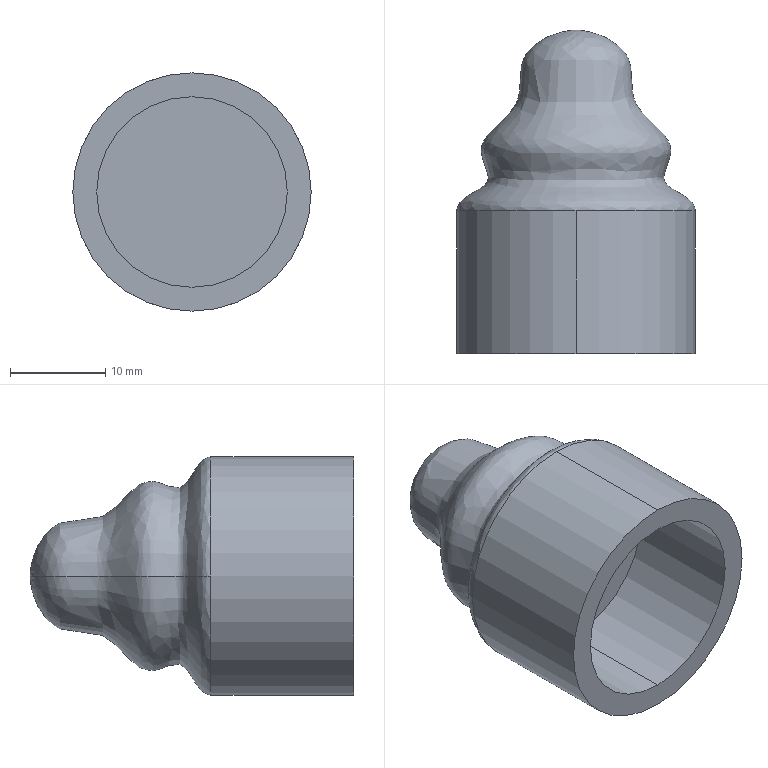Component | SolidWorks | TopCover-1 | 1 solid | 8 faces | box 25 x 33.95 x 25 mm | volume 7353 mm3 | cylinder 4 | spline 2 | plane 2 | commonest cylinder face diameters 20 x2 25 x2
build123d program:
from build123d import *

# Parameters (mm, degrees)
SKETCH1_R           = 12.5
BOSS_EXTRUDE1_DEPTH = 15
SHELL1_T            = -2.5


with BuildPart() as part:
    # Sketch1 → Boss-Extrude1 (new body)
    with BuildSketch(Plane(origin=(0, 0, 0), x_dir=(1, 0, 0), z_dir=(0, 1, 0))):
        with Locations(Location((0, 0, 0), (0, 0, 270))):
            Circle(SKETCH1_R)
    extrude(amount=BOSS_EXTRUDE1_DEPTH)

    # Shell1
    shell1_openings = [part.faces().sort_by_distance(p)[0] for p in [
        (0, 0, 0),
    ]]
    offset(amount=SHELL1_T, openings=shell1_openings, kind=Kind.INTERSECTION)

    # Sketch2 → Revolve1 (revolve)
    with BuildSketch(Plane.XY):
        with BuildLine():
            Line((-12.5, 15), (0, 15))
            Line((0, 15), (0, 33.954))
            add(Edge.make_bspline(
                [(-12.5, 15), (-12.5, 16.591), (-7.793, 17.261), (-11.573, 22.581), (-4.955, 25.26), (-6.75, 32.024), (-1.878, 33.951), (0, 33.954)],
                knots=[0, 0, 0, 0, 0.1825, 0.2981, 0.5567, 0.738, 1, 1, 1, 1], degree=3))
        make_face()
    revolve(axis=Axis((0, 15, 0), (0, 1, 0)))


solid = part.part

# Placed as in the assembly
solid = solid.moved(Location((155, 1577.501, -154.999), (0, 0, 0)))
STEP:
#1=CARTESIAN_POINT('',(6.102,63.443,-6.102));
#2=VERTEX_POINT('',#1);
#3=CARTESIAN_POINT('',(5.61,62.697,-6.102));
#4=VERTEX_POINT('',#3);
#5=CARTESIAN_POINT('',(6.102,63.443,-6.102));
#6=CARTESIAN_POINT('',(6.028,63.443,-6.102));
#7=CARTESIAN_POINT('',(5.837,63.367,-6.102));
#8=CARTESIAN_POINT('',(5.907,63.101,-6.102));
#9=CARTESIAN_POINT('',(5.647,62.995,-6.102));
#10=CARTESIAN_POINT('',(5.796,62.786,-6.102));
#11=CARTESIAN_POINT('',(5.61,62.759,-6.102));
#12=CARTESIAN_POINT('',(5.61,62.697,-6.102));
#13=B_SPLINE_CURVE_WITH_KNOTS('',3,(#5,#6,#7,#8,#9,#10,#11,#12),.UNSPECIFIED.,.F.,.F.,(4,1,1,1,1,4),(0.,0.262,0.4433,0.7019,0.8175,1.),.UNSPECIFIED.);
#14=EDGE_CURVE('',#2,#4,#13,.T.);
#15=ORIENTED_EDGE('',*,*,#14,.F.);
#16=CARTESIAN_POINT('',(6.594,62.697,-6.102));
#17=VERTEX_POINT('',#16);
#18=CARTESIAN_POINT('',(6.102,63.443,-6.102));
#19=CARTESIAN_POINT('',(6.176,63.443,-6.102));
#20=CARTESIAN_POINT('',(6.368,63.367,-6.102));
#21=CARTESIAN_POINT('',(6.297,63.101,-6.102));
#22=CARTESIAN_POINT('',(6.558,62.995,-6.102));
#23=CARTESIAN_POINT('',(6.409,62.786,-6.102));
#24=CARTESIAN_POINT('',(6.594,62.759,-6.102));
#25=CARTESIAN_POINT('',(6.594,62.697,-6.102));
#26=B_SPLINE_CURVE_WITH_KNOTS('',3,(#18,#19,#20,#21,#22,#23,#24,#25),.UNSPECIFIED.,.F.,.F.,(4,1,1,1,1,4),(0.,0.262,0.4433,0.7019,0.8175,1.),.UNSPECIFIED.);
#27=EDGE_CURVE('',#2,#17,#26,.T.);
#28=ORIENTED_EDGE('',*,*,#27,.T.);
#29=CARTESIAN_POINT('',(6.102,62.697,-6.594));
#30=VERTEX_POINT('',#29);
#31=CARTESIAN_POINT('',(6.102,62.697,-6.102));
#32=DIRECTION('',(0.,1.,0.));
#33=DIRECTION('',(0.,0.,1.));
#34=AXIS2_PLACEMENT_3D('',#31,#32,#33);
#35=CIRCLE('',#34,0.4921);
#36=EDGE_CURVE('',#17,#30,#35,.T.);
#37=ORIENTED_EDGE('',*,*,#36,.T.);
#38=CARTESIAN_POINT('',(6.102,62.697,-6.102));
#39=DIRECTION('',(0.,1.,0.));
#40=DIRECTION('',(0.,0.,1.));
#41=AXIS2_PLACEMENT_3D('',#38,#39,#40);
#42=CIRCLE('',#41,0.4921);
#43=EDGE_CURVE('',#30,#4,#42,.T.);
#44=ORIENTED_EDGE('',*,*,#43,.T.);
#45=EDGE_LOOP('',(#15,#28,#37,#44));
#46=FACE_OUTER_BOUND('',#45,.T.);
#47=CARTESIAN_POINT('',(6.102,63.443,-6.102));
#48=CARTESIAN_POINT('',(6.102,63.443,-6.102));
#49=CARTESIAN_POINT('',(6.102,63.443,-6.102));
#50=CARTESIAN_POINT('',(6.102,63.443,-6.102));
#51=CARTESIAN_POINT('',(6.028,63.443,-6.102));
#52=CARTESIAN_POINT('',(6.028,63.443,-6.25));
#53=CARTESIAN_POINT('',(6.176,63.443,-6.25));
#54=CARTESIAN_POINT('',(6.176,63.443,-6.102));
#55=CARTESIAN_POINT('',(5.837,63.367,-6.102));
#56=CARTESIAN_POINT('',(5.837,63.367,-6.634));
#57=CARTESIAN_POINT('',(6.368,63.367,-6.634));
#58=CARTESIAN_POINT('',(6.368,63.367,-6.102));
#59=CARTESIAN_POINT('',(5.907,63.101,-6.102));
#60=CARTESIAN_POINT('',(5.907,63.101,-6.492));
#61=CARTESIAN_POINT('',(6.297,63.101,-6.492));
#62=CARTESIAN_POINT('',(6.297,63.101,-6.102));
#63=CARTESIAN_POINT('',(5.647,62.995,-6.102));
#64=CARTESIAN_POINT('',(5.647,62.995,-7.014));
#65=CARTESIAN_POINT('',(6.558,62.995,-7.014));
#66=CARTESIAN_POINT('',(6.558,62.995,-6.102));
#67=CARTESIAN_POINT('',(5.796,62.786,-6.102));
#68=CARTESIAN_POINT('',(5.796,62.786,-6.716));
#69=CARTESIAN_POINT('',(6.409,62.786,-6.716));
#70=CARTESIAN_POINT('',(6.409,62.786,-6.102));
#71=CARTESIAN_POINT('',(5.61,62.759,-6.102));
#72=CARTESIAN_POINT('',(5.61,62.759,-7.087));
#73=CARTESIAN_POINT('',(6.594,62.759,-7.087));
#74=CARTESIAN_POINT('',(6.594,62.759,-6.102));
#75=CARTESIAN_POINT('',(5.61,62.697,-6.102));
#76=CARTESIAN_POINT('',(5.61,62.697,-7.087));
#77=CARTESIAN_POINT('',(6.594,62.697,-7.087));
#78=CARTESIAN_POINT('',(6.594,62.697,-6.102));
#79=(BOUNDED_SURFACE()B_SPLINE_SURFACE(3,3,((#47,#48,#49,#50),(#51,#52,#53,#54),(#55,#56,#57,#58),(#59,#60,#61,#62),(#63,#64,#65,#66),(#67,#68,#69,#70),(#71,#72,#73,#74),(#75,#76,#77,#78)),.UNSPECIFIED.,.F.,.F.,.T.)B_SPLINE_SURFACE_WITH_KNOTS((4,1,1,1,1,4),(4,4),(0.,0.262,0.4433,0.7019,0.8175,1.),(0.,1.),.UNSPECIFIED.)GEOMETRIC_REPRESENTATION_ITEM()RATIONAL_B_SPLINE_SURFACE(((1.,0.3333,0.3333,1.),(1.,0.3333,0.3333,1.),(1.,0.3333,0.3333,1.),(1.,0.3333,0.3333,1.),(1.,0.3333,0.3333,1.),(1.,0.3333,0.3333,1.),(1.,0.3333,0.3333,1.),(1.,0.3333,0.3333,1.)))REPRESENTATION_ITEM('')SURFACE());
#80=ADVANCED_FACE('',(#46),#79,.F.);
#81=CARTESIAN_POINT('',(6.102,62.598,-6.496));
#82=VERTEX_POINT('',#81);
#83=CARTESIAN_POINT('',(6.102,62.598,-5.709));
#84=VERTEX_POINT('',#83);
#85=CARTESIAN_POINT('',(6.102,62.598,-6.102));
#86=DIRECTION('',(0.,1.,0.));
#87=DIRECTION('',(0.,0.,1.));
#88=AXIS2_PLACEMENT_3D('',#85,#86,#87);
#89=CIRCLE('',#88,0.3937);
#90=EDGE_CURVE('',#82,#84,#89,.T.);
#91=ORIENTED_EDGE('',*,*,#90,.T.);
#92=CARTESIAN_POINT('',(6.102,62.106,-5.709));
#93=VERTEX_POINT('',#92);
#94=CARTESIAN_POINT('',(6.102,62.697,-5.709));
#95=DIRECTION('',(0.,-1.,0.));
#96=VECTOR('',#95,39.37);
#97=LINE('',#94,#96);
#98=EDGE_CURVE('',#84,#93,#97,.T.);
#99=ORIENTED_EDGE('',*,*,#98,.T.);
#100=CARTESIAN_POINT('',(6.102,62.106,-6.496));
#101=VERTEX_POINT('',#100);
#102=CARTESIAN_POINT('',(6.102,62.106,-6.102));
#103=DIRECTION('',(0.,1.,0.));
#104=DIRECTION('',(0.,0.,1.));
#105=AXIS2_PLACEMENT_3D('',#102,#103,#104);
#106=CIRCLE('',#105,0.3937);
#107=EDGE_CURVE('',#101,#93,#106,.T.);
#108=ORIENTED_EDGE('',*,*,#107,.F.);
#109=CARTESIAN_POINT('',(6.102,62.697,-6.496));
#110=DIRECTION('',(0.,-1.,0.));
#111=VECTOR('',#110,39.37);
#112=LINE('',#109,#111);
#113=EDGE_CURVE('',#82,#101,#112,.T.);
#114=ORIENTED_EDGE('',*,*,#113,.F.);
#115=EDGE_LOOP('',(#91,#99,#108,#114));
#116=FACE_OUTER_BOUND('',#115,.T.);
#117=CARTESIAN_POINT('',(6.102,62.697,-6.102));
#118=DIRECTION('',(0.,-1.,0.));
#119=DIRECTION('',(0.,0.,-1.));
#120=AXIS2_PLACEMENT_3D('',#117,#118,#119);
#121=CYLINDRICAL_SURFACE('',#120,0.3937);
#122=ADVANCED_FACE('',(#116),#121,.F.);
#123=CARTESIAN_POINT('',(6.102,62.697,-5.61));
#124=VERTEX_POINT('',#123);
#125=CARTESIAN_POINT('',(6.102,62.697,-6.102));
#126=DIRECTION('',(0.,1.,0.));
#127=DIRECTION('',(0.,0.,1.));
#128=AXIS2_PLACEMENT_3D('',#125,#126,#127);
#129=CIRCLE('',#128,0.4921);
#130=EDGE_CURVE('',#124,#17,#129,.T.);
#131=ORIENTED_EDGE('',*,*,#130,.F.);
#132=CARTESIAN_POINT('',(6.102,62.106,-5.61));
#133=VERTEX_POINT('',#132);
#134=CARTESIAN_POINT('',(6.102,62.697,-5.61));
#135=DIRECTION('',(0.,-1.,0.));
#136=VECTOR('',#135,39.37);
#137=LINE('',#134,#136);
#138=EDGE_CURVE('',#124,#133,#137,.T.);
#139=ORIENTED_EDGE('',*,*,#138,.T.);
#140=CARTESIAN_POINT('',(6.102,62.106,-6.594));
#141=VERTEX_POINT('',#140);
#142=CARTESIAN_POINT('',(6.102,62.106,-6.102));
#143=DIRECTION('',(0.,1.,0.));
#144=DIRECTION('',(0.,0.,1.));
#145=AXIS2_PLACEMENT_3D('',#142,#143,#144);
#146=CIRCLE('',#145,0.4921);
#147=EDGE_CURVE('',#133,#141,#146,.T.);
#148=ORIENTED_EDGE('',*,*,#147,.T.);
#149=CARTESIAN_POINT('',(6.102,62.697,-6.594));
#150=DIRECTION('',(0.,-1.,0.));
#151=VECTOR('',#150,39.37);
#152=LINE('',#149,#151);
#153=EDGE_CURVE('',#30,#141,#152,.T.);
#154=ORIENTED_EDGE('',*,*,#153,.F.);
#155=ORIENTED_EDGE('',*,*,#36,.F.);
#156=EDGE_LOOP('',(#131,#139,#148,#154,#155));
#157=FACE_OUTER_BOUND('',#156,.T.);
#158=CARTESIAN_POINT('',(6.102,62.697,-6.102));
#159=DIRECTION('',(0.,-1.,0.));
#160=DIRECTION('',(0.,0.,-1.));
#161=AXIS2_PLACEMENT_3D('',#158,#159,#160);
#162=CYLINDRICAL_SURFACE('',#161,0.4921);
#163=ADVANCED_FACE('',(#157),#162,.T.);
#164=ORIENTED_EDGE('',*,*,#138,.F.);
#165=CARTESIAN_POINT('',(6.102,62.697,-6.102));
#166=DIRECTION('',(0.,1.,0.));
#167=DIRECTION('',(0.,0.,1.));
#168=AXIS2_PLACEMENT_3D('',#165,#166,#167);
#169=CIRCLE('',#168,0.4921);
#170=EDGE_CURVE('',#4,#124,#169,.T.);
#171=ORIENTED_EDGE('',*,*,#170,.F.);
#172=ORIENTED_EDGE('',*,*,#43,.F.);
#173=ORIENTED_EDGE('',*,*,#153,.T.);
#174=CARTESIAN_POINT('',(6.102,62.106,-6.102));
#175=DIRECTION('',(0.,1.,0.));
#176=DIRECTION('',(0.,0.,1.));
#177=AXIS2_PLACEMENT_3D('',#174,#175,#176);
#178=CIRCLE('',#177,0.4921);
#179=EDGE_CURVE('',#141,#133,#178,.T.);
#180=ORIENTED_EDGE('',*,*,#179,.T.);
#181=EDGE_LOOP('',(#164,#171,#172,#173,#180));
#182=FACE_OUTER_BOUND('',#181,.T.);
#183=CARTESIAN_POINT('',(6.102,62.697,-6.102));
#184=DIRECTION('',(0.,-1.,0.));
#185=DIRECTION('',(0.,0.,-1.));
#186=AXIS2_PLACEMENT_3D('',#183,#184,#185);
#187=CYLINDRICAL_SURFACE('',#186,0.4921);
#188=ADVANCED_FACE('',(#182),#187,.T.);
#189=ORIENTED_EDGE('',*,*,#107,.T.);
#190=CARTESIAN_POINT('',(6.102,62.106,-6.102));
#191=DIRECTION('',(0.,1.,0.));
#192=DIRECTION('',(0.,0.,1.));
#193=AXIS2_PLACEMENT_3D('',#190,#191,#192);
#194=CIRCLE('',#193,0.3937);
#195=EDGE_CURVE('',#93,#101,#194,.T.);
#196=ORIENTED_EDGE('',*,*,#195,.T.);
#197=EDGE_LOOP('',(#189,#196));
#198=FACE_BOUND('',#197,.T.);
#199=ORIENTED_EDGE('',*,*,#179,.F.);
#200=ORIENTED_EDGE('',*,*,#147,.F.);
#201=EDGE_LOOP('',(#199,#200));
#202=FACE_OUTER_BOUND('',#201,.T.);
#203=CARTESIAN_POINT('',(6.102,62.106,-6.102));
#204=DIRECTION('',(0.,1.,0.));
#205=DIRECTION('',(0.,0.,1.));
#206=AXIS2_PLACEMENT_3D('',#203,#204,#205);
#207=PLANE('',#206);
#208=ADVANCED_FACE('',(#198,#202),#207,.F.);
#209=ORIENTED_EDGE('',*,*,#98,.F.);
#210=CARTESIAN_POINT('',(6.102,62.598,-6.102));
#211=DIRECTION('',(0.,1.,0.));
#212=DIRECTION('',(0.,0.,1.));
#213=AXIS2_PLACEMENT_3D('',#210,#211,#212);
#214=CIRCLE('',#213,0.3937);
#215=EDGE_CURVE('',#84,#82,#214,.T.);
#216=ORIENTED_EDGE('',*,*,#215,.T.);
#217=ORIENTED_EDGE('',*,*,#113,.T.);
#218=ORIENTED_EDGE('',*,*,#195,.F.);
#219=EDGE_LOOP('',(#209,#216,#217,#218));
#220=FACE_OUTER_BOUND('',#219,.T.);
#221=CARTESIAN_POINT('',(6.102,62.697,-6.102));
#222=DIRECTION('',(0.,-1.,0.));
#223=DIRECTION('',(0.,0.,-1.));
#224=AXIS2_PLACEMENT_3D('',#221,#222,#223);
#225=CYLINDRICAL_SURFACE('',#224,0.3937);
#226=ADVANCED_FACE('',(#220),#225,.F.);
#227=ORIENTED_EDGE('',*,*,#90,.F.);
#228=ORIENTED_EDGE('',*,*,#215,.F.);
#229=EDGE_LOOP('',(#227,#228));
#230=FACE_OUTER_BOUND('',#229,.T.);
#231=CARTESIAN_POINT('',(6.102,62.598,-6.102));
#232=DIRECTION('',(0.,1.,0.));
#233=DIRECTION('',(0.,0.,1.));
#234=AXIS2_PLACEMENT_3D('',#231,#232,#233);
#235=PLANE('',#234);
#236=ADVANCED_FACE('',(#230),#235,.F.);
#237=ORIENTED_EDGE('',*,*,#27,.F.);
#238=ORIENTED_EDGE('',*,*,#14,.T.);
#239=ORIENTED_EDGE('',*,*,#170,.T.);
#240=ORIENTED_EDGE('',*,*,#130,.T.);
#241=EDGE_LOOP('',(#237,#238,#239,#240));
#242=FACE_OUTER_BOUND('',#241,.T.);
#243=CARTESIAN_POINT('',(6.102,63.443,-6.102));
#244=CARTESIAN_POINT('',(6.102,63.443,-6.102));
#245=CARTESIAN_POINT('',(6.102,63.443,-6.102));
#246=CARTESIAN_POINT('',(6.102,63.443,-6.102));
#247=CARTESIAN_POINT('',(6.176,63.443,-6.102));
#248=CARTESIAN_POINT('',(6.176,63.443,-5.954));
#249=CARTESIAN_POINT('',(6.028,63.443,-5.954));
#250=CARTESIAN_POINT('',(6.028,63.443,-6.102));
#251=CARTESIAN_POINT('',(6.368,63.367,-6.102));
#252=CARTESIAN_POINT('',(6.368,63.367,-5.571));
#253=CARTESIAN_POINT('',(5.837,63.367,-5.571));
#254=CARTESIAN_POINT('',(5.837,63.367,-6.102));
#255=CARTESIAN_POINT('',(6.297,63.101,-6.102));
#256=CARTESIAN_POINT('',(6.297,63.101,-5.712));
#257=CARTESIAN_POINT('',(5.907,63.101,-5.712));
#258=CARTESIAN_POINT('',(5.907,63.101,-6.102));
#259=CARTESIAN_POINT('',(6.558,62.995,-6.102));
#260=CARTESIAN_POINT('',(6.558,62.995,-5.191));
#261=CARTESIAN_POINT('',(5.647,62.995,-5.191));
#262=CARTESIAN_POINT('',(5.647,62.995,-6.102));
#263=CARTESIAN_POINT('',(6.409,62.786,-6.102));
#264=CARTESIAN_POINT('',(6.409,62.786,-5.489));
#265=CARTESIAN_POINT('',(5.796,62.786,-5.489));
#266=CARTESIAN_POINT('',(5.796,62.786,-6.102));
#267=CARTESIAN_POINT('',(6.594,62.759,-6.102));
#268=CARTESIAN_POINT('',(6.594,62.759,-5.118));
#269=CARTESIAN_POINT('',(5.61,62.759,-5.118));
#270=CARTESIAN_POINT('',(5.61,62.759,-6.102));
#271=CARTESIAN_POINT('',(6.594,62.697,-6.102));
#272=CARTESIAN_POINT('',(6.594,62.697,-5.118));
#273=CARTESIAN_POINT('',(5.61,62.697,-5.118));
#274=CARTESIAN_POINT('',(5.61,62.697,-6.102));
#275=(BOUNDED_SURFACE()B_SPLINE_SURFACE(3,3,((#243,#244,#245,#246),(#247,#248,#249,#250),(#251,#252,#253,#254),(#255,#256,#257,#258),(#259,#260,#261,#262),(#263,#264,#265,#266),(#267,#268,#269,#270),(#271,#272,#273,#274)),.UNSPECIFIED.,.F.,.F.,.T.)B_SPLINE_SURFACE_WITH_KNOTS((4,1,1,1,1,4),(4,4),(0.,0.262,0.4433,0.7019,0.8175,1.),(0.,1.),.UNSPECIFIED.)GEOMETRIC_REPRESENTATION_ITEM()RATIONAL_B_SPLINE_SURFACE(((1.,0.3333,0.3333,1.),(1.,0.3333,0.3333,1.),(1.,0.3333,0.3333,1.),(1.,0.3333,0.3333,1.),(1.,0.3333,0.3333,1.),(1.,0.3333,0.3333,1.),(1.,0.3333,0.3333,1.),(1.,0.3333,0.3333,1.)))REPRESENTATION_ITEM('')SURFACE());
#276=ADVANCED_FACE('',(#242),#275,.F.);
#277=CLOSED_SHELL('',(#80,#122,#163,#188,#208,#226,#236,#276));
#278=MANIFOLD_SOLID_BREP('',#277);
#279=CARTESIAN_POINT('',(0.,0.,0.));
#280=DIRECTION('',(0.,0.,1.));
#281=DIRECTION('',(1.,0.,0.));
#282=AXIS2_PLACEMENT_3D('',#279,#280,#281);
#283=(LENGTH_UNIT()NAMED_UNIT(*)SI_UNIT($,.METRE.));
#284=LENGTH_MEASURE_WITH_UNIT(LENGTH_MEASURE(0.0254),#283);
#285=DIMENSIONAL_EXPONENTS(1.,0.,0.,0.,0.,0.,0.);
#286=(CONVERSION_BASED_UNIT('',#284)LENGTH_UNIT()NAMED_UNIT(#285));
#287=UNCERTAINTY_MEASURE_WITH_UNIT(LENGTH_MEASURE(0.00001),#286,'','');
#288=(NAMED_UNIT(*)PLANE_ANGLE_UNIT()SI_UNIT($,.RADIAN.));
#289=(NAMED_UNIT(*)SI_UNIT($,.STERADIAN.)SOLID_ANGLE_UNIT());
#290=(GEOMETRIC_REPRESENTATION_CONTEXT(3)GLOBAL_UNCERTAINTY_ASSIGNED_CONTEXT((#287))GLOBAL_UNIT_ASSIGNED_CONTEXT((#286,#288,#289))REPRESENTATION_CONTEXT('',''));
#291=ADVANCED_BREP_SHAPE_REPRESENTATION('',(#278,#282),#290);
#292=COLOUR_RGB('',0.7922,0.8196,0.9333);
#293=FILL_AREA_STYLE_COLOUR('',#292);
#294=FILL_AREA_STYLE('',(#293));
#295=SURFACE_STYLE_FILL_AREA(#294);
#296=SURFACE_SIDE_STYLE('',(#295));
#297=SURFACE_STYLE_USAGE(.BOTH.,#296);
#298=PRESENTATION_STYLE_ASSIGNMENT((#297));
#299=STYLED_ITEM('',(#298),#278);
#300=(LENGTH_UNIT()NAMED_UNIT(*)SI_UNIT($,.METRE.));
#301=LENGTH_MEASURE_WITH_UNIT(LENGTH_MEASURE(0.0254),#300);
#302=DIMENSIONAL_EXPONENTS(1.,0.,0.,0.,0.,0.,0.);
#303=(CONVERSION_BASED_UNIT('',#301)LENGTH_UNIT()NAMED_UNIT(#302));
#304=UNCERTAINTY_MEASURE_WITH_UNIT(LENGTH_MEASURE(0.00001),#303,'','');
#305=(NAMED_UNIT(*)PLANE_ANGLE_UNIT()SI_UNIT($,.RADIAN.));
#306=(NAMED_UNIT(*)SI_UNIT($,.STERADIAN.)SOLID_ANGLE_UNIT());
#307=(GEOMETRIC_REPRESENTATION_CONTEXT(3)GLOBAL_UNCERTAINTY_ASSIGNED_CONTEXT((#304))GLOBAL_UNIT_ASSIGNED_CONTEXT((#303,#305,#306))REPRESENTATION_CONTEXT('',''));
#308=MECHANICAL_DESIGN_GEOMETRIC_PRESENTATION_REPRESENTATION('',(#299),#307);
#309=PRESENTATION_LAYER_ASSIGNMENT('','',(#299));